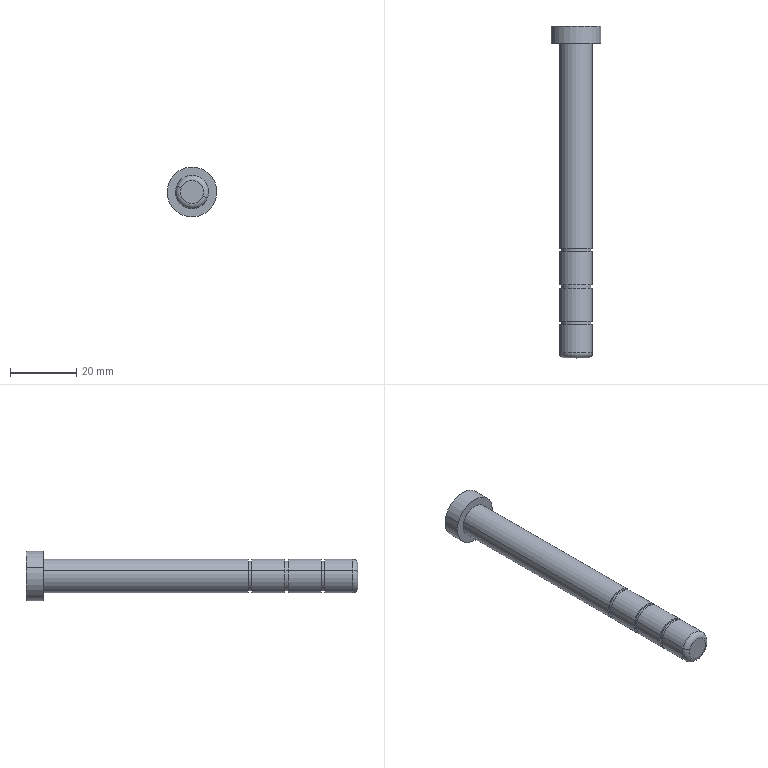Component | SolidWorks | GP-10-100-2GuidePin-2 | 1 solid | 27 faces | box 15 x 100 x 15 mm | volume 8306 mm3 | cylinder 16 | plane 9 | torus 2 | commonest cylinder face diameters 10 x8 9 x6 15 x2
build123d program:
from build123d import *

# Parameters (mm, degrees)
FILLET1_R = 1.5


with BuildPart() as part:
    # Sketch1 → Revolve1 (revolve)
    with BuildSketch(Plane.XY, mode=Mode.PRIVATE) as revolve1_sk:
        Polygon((0, 100), (5, 100), (5, 90), (4.5, 90), (4.5, 89), (5, 89), (5, 79), (4.5, 79), (4.5, 78), (5, 78), (5, 68), (4.5, 68), (4.5, 67), (5, 67), (5, 5.2), (7.5, 5.2), (7.5, 0), (0, 0), align=None)
    revolve(revolve1_sk.sketch.rotate(Axis((0, 100, 0), (0, -1, 0)), 180), axis=Axis((0, 100, 0), (0, -1, 0)))

    # Fillet1
    fillet1_edges = [part.edges().sort_by_distance(p)[0] for p in [
        (5, 100, 0),
    ]]
    fillet(fillet1_edges, radius=FILLET1_R)


solid = part.part

# Placed as in the assembly
solid = solid.moved(Location((139.884, -65.161, 270), (180, 0, 0)))
STEP:
#1=CARTESIAN_POINT('',(5.378,-6.502,10.677));
#2=VERTEX_POINT('',#1);
#3=CARTESIAN_POINT('',(5.637,-6.502,10.583));
#4=VERTEX_POINT('',#3);
#5=CARTESIAN_POINT('',(5.507,-6.502,10.63));
#6=DIRECTION('',(-0.,-1.,0.));
#7=DIRECTION('',(0.9396,0.,-0.3423));
#8=AXIS2_PLACEMENT_3D('',#5,#6,#7);
#9=CIRCLE('',#8,0.1378);
#10=EDGE_CURVE('',#2,#4,#9,.T.);
#11=ORIENTED_EDGE('',*,*,#10,.F.);
#12=CARTESIAN_POINT('',(5.322,-6.443,10.697));
#13=VERTEX_POINT('',#12);
#14=CARTESIAN_POINT('',(5.378,-6.443,10.677));
#15=DIRECTION('',(-0.3423,0.,-0.9396));
#16=DIRECTION('',(-0.9396,0.,0.3423));
#17=AXIS2_PLACEMENT_3D('',#14,#15,#16);
#18=CIRCLE('',#17,0.05906);
#19=EDGE_CURVE('',#2,#13,#18,.T.);
#20=ORIENTED_EDGE('',*,*,#19,.T.);
#21=CARTESIAN_POINT('',(5.692,-6.443,10.563));
#22=VERTEX_POINT('',#21);
#23=CARTESIAN_POINT('',(5.507,-6.443,10.63));
#24=DIRECTION('',(0.,1.,-0.));
#25=DIRECTION('',(0.9396,0.,-0.3423));
#26=AXIS2_PLACEMENT_3D('',#23,#24,#25);
#27=CIRCLE('',#26,0.1969);
#28=EDGE_CURVE('',#22,#13,#27,.T.);
#29=ORIENTED_EDGE('',*,*,#28,.F.);
#30=CARTESIAN_POINT('',(5.637,-6.443,10.583));
#31=DIRECTION('',(0.3423,-0.,0.9396));
#32=DIRECTION('',(0.9396,0.,-0.3423));
#33=AXIS2_PLACEMENT_3D('',#30,#31,#32);
#34=CIRCLE('',#33,0.05906);
#35=EDGE_CURVE('',#4,#22,#34,.T.);
#36=ORIENTED_EDGE('',*,*,#35,.F.);
#37=EDGE_LOOP('',(#11,#20,#29,#36));
#38=FACE_OUTER_BOUND('',#37,.T.);
#39=CARTESIAN_POINT('',(5.507,-6.443,10.63));
#40=DIRECTION('',(0.,1.,-0.));
#41=DIRECTION('',(0.9396,-0.,-0.3423));
#42=AXIS2_PLACEMENT_3D('',#39,#40,#41);
#43=TOROIDAL_SURFACE('',#42,0.1378,0.05906);
#44=ADVANCED_FACE('',(#38),#43,.T.);
#45=CARTESIAN_POINT('',(5.23,-2.565,10.731));
#46=VERTEX_POINT('',#45);
#47=CARTESIAN_POINT('',(5.785,-2.565,10.529));
#48=VERTEX_POINT('',#47);
#49=CARTESIAN_POINT('',(5.507,-2.565,10.63));
#50=DIRECTION('',(-0.,-1.,0.));
#51=DIRECTION('',(-0.9396,0.,0.3423));
#52=AXIS2_PLACEMENT_3D('',#49,#50,#51);
#53=CIRCLE('',#52,0.2953);
#54=EDGE_CURVE('',#46,#48,#53,.T.);
#55=ORIENTED_EDGE('',*,*,#54,.T.);
#56=CARTESIAN_POINT('',(5.785,-2.77,10.529));
#57=VERTEX_POINT('',#56);
#58=CARTESIAN_POINT('',(5.785,-6.502,10.529));
#59=DIRECTION('',(-0.,-1.,0.));
#60=VECTOR('',#59,39.37);
#61=LINE('',#58,#60);
#62=EDGE_CURVE('',#48,#57,#61,.T.);
#63=ORIENTED_EDGE('',*,*,#62,.T.);
#64=CARTESIAN_POINT('',(5.23,-2.77,10.731));
#65=VERTEX_POINT('',#64);
#66=CARTESIAN_POINT('',(5.507,-2.77,10.63));
#67=DIRECTION('',(-0.,-1.,0.));
#68=DIRECTION('',(-0.9396,0.,0.3423));
#69=AXIS2_PLACEMENT_3D('',#66,#67,#68);
#70=CIRCLE('',#69,0.2953);
#71=EDGE_CURVE('',#65,#57,#70,.T.);
#72=ORIENTED_EDGE('',*,*,#71,.F.);
#73=CARTESIAN_POINT('',(5.23,-6.502,10.731));
#74=DIRECTION('',(-0.,-1.,0.));
#75=VECTOR('',#74,39.37);
#76=LINE('',#73,#75);
#77=EDGE_CURVE('',#46,#65,#76,.T.);
#78=ORIENTED_EDGE('',*,*,#77,.F.);
#79=EDGE_LOOP('',(#55,#63,#72,#78));
#80=FACE_OUTER_BOUND('',#79,.T.);
#81=CARTESIAN_POINT('',(5.507,-6.502,10.63));
#82=DIRECTION('',(-0.,-1.,0.));
#83=DIRECTION('',(-0.9396,0.,0.3423));
#84=AXIS2_PLACEMENT_3D('',#81,#82,#83);
#85=CYLINDRICAL_SURFACE('',#84,0.2953);
#86=ADVANCED_FACE('',(#80),#85,.T.);
#87=CARTESIAN_POINT('',(5.322,-2.77,10.697));
#88=VERTEX_POINT('',#87);
#89=CARTESIAN_POINT('',(5.692,-2.77,10.563));
#90=VERTEX_POINT('',#89);
#91=CARTESIAN_POINT('',(5.507,-2.77,10.63));
#92=DIRECTION('',(-0.,-1.,0.));
#93=DIRECTION('',(-0.9396,0.,0.3423));
#94=AXIS2_PLACEMENT_3D('',#91,#92,#93);
#95=CIRCLE('',#94,0.1969);
#96=EDGE_CURVE('',#88,#90,#95,.T.);
#97=ORIENTED_EDGE('',*,*,#96,.T.);
#98=CARTESIAN_POINT('',(5.692,-5.203,10.563));
#99=VERTEX_POINT('',#98);
#100=CARTESIAN_POINT('',(5.692,-6.502,10.563));
#101=DIRECTION('',(-0.,-1.,0.));
#102=VECTOR('',#101,39.37);
#103=LINE('',#100,#102);
#104=EDGE_CURVE('',#90,#99,#103,.T.);
#105=ORIENTED_EDGE('',*,*,#104,.T.);
#106=CARTESIAN_POINT('',(5.322,-5.203,10.697));
#107=VERTEX_POINT('',#106);
#108=CARTESIAN_POINT('',(5.507,-5.203,10.63));
#109=DIRECTION('',(-0.,-1.,0.));
#110=DIRECTION('',(-0.9396,0.,0.3423));
#111=AXIS2_PLACEMENT_3D('',#108,#109,#110);
#112=CIRCLE('',#111,0.1969);
#113=EDGE_CURVE('',#107,#99,#112,.T.);
#114=ORIENTED_EDGE('',*,*,#113,.F.);
#115=CARTESIAN_POINT('',(5.322,-6.502,10.697));
#116=DIRECTION('',(-0.,-1.,0.));
#117=VECTOR('',#116,39.37);
#118=LINE('',#115,#117);
#119=EDGE_CURVE('',#88,#107,#118,.T.);
#120=ORIENTED_EDGE('',*,*,#119,.F.);
#121=EDGE_LOOP('',(#97,#105,#114,#120));
#122=FACE_OUTER_BOUND('',#121,.T.);
#123=CARTESIAN_POINT('',(5.507,-6.502,10.63));
#124=DIRECTION('',(-0.,-1.,0.));
#125=DIRECTION('',(-0.9396,0.,0.3423));
#126=AXIS2_PLACEMENT_3D('',#123,#124,#125);
#127=CYLINDRICAL_SURFACE('',#126,0.1969);
#128=ADVANCED_FACE('',(#122),#127,.T.);
#129=CARTESIAN_POINT('',(5.341,-5.203,10.691));
#130=VERTEX_POINT('',#129);
#131=CARTESIAN_POINT('',(5.674,-5.203,10.569));
#132=VERTEX_POINT('',#131);
#133=CARTESIAN_POINT('',(5.507,-5.203,10.63));
#134=DIRECTION('',(-0.,-1.,0.));
#135=DIRECTION('',(-0.9396,0.,0.3423));
#136=AXIS2_PLACEMENT_3D('',#133,#134,#135);
#137=CIRCLE('',#136,0.1772);
#138=EDGE_CURVE('',#130,#132,#137,.T.);
#139=ORIENTED_EDGE('',*,*,#138,.T.);
#140=CARTESIAN_POINT('',(5.674,-5.243,10.569));
#141=VERTEX_POINT('',#140);
#142=CARTESIAN_POINT('',(5.674,-6.502,10.569));
#143=DIRECTION('',(-0.,-1.,0.));
#144=VECTOR('',#143,39.37);
#145=LINE('',#142,#144);
#146=EDGE_CURVE('',#132,#141,#145,.T.);
#147=ORIENTED_EDGE('',*,*,#146,.T.);
#148=CARTESIAN_POINT('',(5.341,-5.243,10.691));
#149=VERTEX_POINT('',#148);
#150=CARTESIAN_POINT('',(5.507,-5.243,10.63));
#151=DIRECTION('',(-0.,-1.,0.));
#152=DIRECTION('',(-0.9396,0.,0.3423));
#153=AXIS2_PLACEMENT_3D('',#150,#151,#152);
#154=CIRCLE('',#153,0.1772);
#155=EDGE_CURVE('',#149,#141,#154,.T.);
#156=ORIENTED_EDGE('',*,*,#155,.F.);
#157=CARTESIAN_POINT('',(5.341,-6.502,10.691));
#158=DIRECTION('',(-0.,-1.,0.));
#159=VECTOR('',#158,39.37);
#160=LINE('',#157,#159);
#161=EDGE_CURVE('',#130,#149,#160,.T.);
#162=ORIENTED_EDGE('',*,*,#161,.F.);
#163=EDGE_LOOP('',(#139,#147,#156,#162));
#164=FACE_OUTER_BOUND('',#163,.T.);
#165=CARTESIAN_POINT('',(5.507,-6.502,10.63));
#166=DIRECTION('',(-0.,-1.,0.));
#167=DIRECTION('',(-0.9396,0.,0.3423));
#168=AXIS2_PLACEMENT_3D('',#165,#166,#167);
#169=CYLINDRICAL_SURFACE('',#168,0.1772);
#170=ADVANCED_FACE('',(#164),#169,.T.);
#171=CARTESIAN_POINT('',(5.322,-5.243,10.697));
#172=VERTEX_POINT('',#171);
#173=CARTESIAN_POINT('',(5.692,-5.243,10.563));
#174=VERTEX_POINT('',#173);
#175=CARTESIAN_POINT('',(5.507,-5.243,10.63));
#176=DIRECTION('',(-0.,-1.,0.));
#177=DIRECTION('',(-0.9396,0.,0.3423));
#178=AXIS2_PLACEMENT_3D('',#175,#176,#177);
#179=CIRCLE('',#178,0.1969);
#180=EDGE_CURVE('',#172,#174,#179,.T.);
#181=ORIENTED_EDGE('',*,*,#180,.T.);
#182=CARTESIAN_POINT('',(5.692,-5.636,10.563));
#183=VERTEX_POINT('',#182);
#184=CARTESIAN_POINT('',(5.692,-6.502,10.563));
#185=DIRECTION('',(-0.,-1.,0.));
#186=VECTOR('',#185,39.37);
#187=LINE('',#184,#186);
#188=EDGE_CURVE('',#174,#183,#187,.T.);
#189=ORIENTED_EDGE('',*,*,#188,.T.);
#190=CARTESIAN_POINT('',(5.322,-5.636,10.697));
#191=VERTEX_POINT('',#190);
#192=CARTESIAN_POINT('',(5.507,-5.636,10.63));
#193=DIRECTION('',(-0.,-1.,0.));
#194=DIRECTION('',(-0.9396,0.,0.3423));
#195=AXIS2_PLACEMENT_3D('',#192,#193,#194);
#196=CIRCLE('',#195,0.1969);
#197=EDGE_CURVE('',#191,#183,#196,.T.);
#198=ORIENTED_EDGE('',*,*,#197,.F.);
#199=CARTESIAN_POINT('',(5.322,-6.502,10.697));
#200=DIRECTION('',(-0.,-1.,0.));
#201=VECTOR('',#200,39.37);
#202=LINE('',#199,#201);
#203=EDGE_CURVE('',#172,#191,#202,.T.);
#204=ORIENTED_EDGE('',*,*,#203,.F.);
#205=EDGE_LOOP('',(#181,#189,#198,#204));
#206=FACE_OUTER_BOUND('',#205,.T.);
#207=CARTESIAN_POINT('',(5.507,-6.502,10.63));
#208=DIRECTION('',(-0.,-1.,0.));
#209=DIRECTION('',(-0.9396,0.,0.3423));
#210=AXIS2_PLACEMENT_3D('',#207,#208,#209);
#211=CYLINDRICAL_SURFACE('',#210,0.1969);
#212=ADVANCED_FACE('',(#206),#211,.T.);
#213=CARTESIAN_POINT('',(5.341,-5.636,10.691));
#214=VERTEX_POINT('',#213);
#215=CARTESIAN_POINT('',(5.674,-5.636,10.569));
#216=VERTEX_POINT('',#215);
#217=CARTESIAN_POINT('',(5.507,-5.636,10.63));
#218=DIRECTION('',(-0.,-1.,0.));
#219=DIRECTION('',(-0.9396,0.,0.3423));
#220=AXIS2_PLACEMENT_3D('',#217,#218,#219);
#221=CIRCLE('',#220,0.1772);
#222=EDGE_CURVE('',#214,#216,#221,.T.);
#223=ORIENTED_EDGE('',*,*,#222,.T.);
#224=CARTESIAN_POINT('',(5.674,-5.676,10.569));
#225=VERTEX_POINT('',#224);
#226=CARTESIAN_POINT('',(5.674,-6.502,10.569));
#227=DIRECTION('',(-0.,-1.,0.));
#228=VECTOR('',#227,39.37);
#229=LINE('',#226,#228);
#230=EDGE_CURVE('',#216,#225,#229,.T.);
#231=ORIENTED_EDGE('',*,*,#230,.T.);
#232=CARTESIAN_POINT('',(5.341,-5.676,10.691));
#233=VERTEX_POINT('',#232);
#234=CARTESIAN_POINT('',(5.507,-5.676,10.63));
#235=DIRECTION('',(-0.,-1.,0.));
#236=DIRECTION('',(-0.9396,0.,0.3423));
#237=AXIS2_PLACEMENT_3D('',#234,#235,#236);
#238=CIRCLE('',#237,0.1772);
#239=EDGE_CURVE('',#233,#225,#238,.T.);
#240=ORIENTED_EDGE('',*,*,#239,.F.);
#241=CARTESIAN_POINT('',(5.341,-6.502,10.691));
#242=DIRECTION('',(-0.,-1.,0.));
#243=VECTOR('',#242,39.37);
#244=LINE('',#241,#243);
#245=EDGE_CURVE('',#214,#233,#244,.T.);
#246=ORIENTED_EDGE('',*,*,#245,.F.);
#247=EDGE_LOOP('',(#223,#231,#240,#246));
#248=FACE_OUTER_BOUND('',#247,.T.);
#249=CARTESIAN_POINT('',(5.507,-6.502,10.63));
#250=DIRECTION('',(-0.,-1.,0.));
#251=DIRECTION('',(-0.9396,0.,0.3423));
#252=AXIS2_PLACEMENT_3D('',#249,#250,#251);
#253=CYLINDRICAL_SURFACE('',#252,0.1772);
#254=ADVANCED_FACE('',(#248),#253,.T.);
#255=CARTESIAN_POINT('',(5.322,-5.676,10.697));
#256=VERTEX_POINT('',#255);
#257=CARTESIAN_POINT('',(5.692,-5.676,10.563));
#258=VERTEX_POINT('',#257);
#259=CARTESIAN_POINT('',(5.507,-5.676,10.63));
#260=DIRECTION('',(-0.,-1.,0.));
#261=DIRECTION('',(-0.9396,0.,0.3423));
#262=AXIS2_PLACEMENT_3D('',#259,#260,#261);
#263=CIRCLE('',#262,0.1969);
#264=EDGE_CURVE('',#256,#258,#263,.T.);
#265=ORIENTED_EDGE('',*,*,#264,.T.);
#266=CARTESIAN_POINT('',(5.692,-6.069,10.563));
#267=VERTEX_POINT('',#266);
#268=CARTESIAN_POINT('',(5.692,-6.502,10.563));
#269=DIRECTION('',(-0.,-1.,0.));
#270=VECTOR('',#269,39.37);
#271=LINE('',#268,#270);
#272=EDGE_CURVE('',#258,#267,#271,.T.);
#273=ORIENTED_EDGE('',*,*,#272,.T.);
#274=CARTESIAN_POINT('',(5.322,-6.069,10.697));
#275=VERTEX_POINT('',#274);
#276=CARTESIAN_POINT('',(5.507,-6.069,10.63));
#277=DIRECTION('',(-0.,-1.,0.));
#278=DIRECTION('',(-0.9396,0.,0.3423));
#279=AXIS2_PLACEMENT_3D('',#276,#277,#278);
#280=CIRCLE('',#279,0.1969);
#281=EDGE_CURVE('',#275,#267,#280,.T.);
#282=ORIENTED_EDGE('',*,*,#281,.F.);
#283=CARTESIAN_POINT('',(5.322,-6.502,10.697));
#284=DIRECTION('',(-0.,-1.,0.));
#285=VECTOR('',#284,39.37);
#286=LINE('',#283,#285);
#287=EDGE_CURVE('',#256,#275,#286,.T.);
#288=ORIENTED_EDGE('',*,*,#287,.F.);
#289=EDGE_LOOP('',(#265,#273,#282,#288));
#290=FACE_OUTER_BOUND('',#289,.T.);
#291=CARTESIAN_POINT('',(5.507,-6.502,10.63));
#292=DIRECTION('',(-0.,-1.,0.));
#293=DIRECTION('',(-0.9396,0.,0.3423));
#294=AXIS2_PLACEMENT_3D('',#291,#292,#293);
#295=CYLINDRICAL_SURFACE('',#294,0.1969);
#296=ADVANCED_FACE('',(#290),#295,.T.);
#297=CARTESIAN_POINT('',(5.341,-6.069,10.691));
#298=VERTEX_POINT('',#297);
#299=CARTESIAN_POINT('',(5.674,-6.069,10.569));
#300=VERTEX_POINT('',#299);
#301=CARTESIAN_POINT('',(5.507,-6.069,10.63));
#302=DIRECTION('',(-0.,-1.,0.));
#303=DIRECTION('',(-0.9396,0.,0.3423));
#304=AXIS2_PLACEMENT_3D('',#301,#302,#303);
#305=CIRCLE('',#304,0.1772);
#306=EDGE_CURVE('',#298,#300,#305,.T.);
#307=ORIENTED_EDGE('',*,*,#306,.T.);
#308=CARTESIAN_POINT('',(5.674,-6.109,10.569));
#309=VERTEX_POINT('',#308);
#310=CARTESIAN_POINT('',(5.674,-6.502,10.569));
#311=DIRECTION('',(-0.,-1.,0.));
#312=VECTOR('',#311,39.37);
#313=LINE('',#310,#312);
#314=EDGE_CURVE('',#300,#309,#313,.T.);
#315=ORIENTED_EDGE('',*,*,#314,.T.);
#316=CARTESIAN_POINT('',(5.341,-6.109,10.691));
#317=VERTEX_POINT('',#316);
#318=CARTESIAN_POINT('',(5.507,-6.109,10.63));
#319=DIRECTION('',(-0.,-1.,0.));
#320=DIRECTION('',(-0.9396,0.,0.3423));
#321=AXIS2_PLACEMENT_3D('',#318,#319,#320);
#322=CIRCLE('',#321,0.1772);
#323=EDGE_CURVE('',#317,#309,#322,.T.);
#324=ORIENTED_EDGE('',*,*,#323,.F.);
#325=CARTESIAN_POINT('',(5.341,-6.502,10.691));
#326=DIRECTION('',(-0.,-1.,0.));
#327=VECTOR('',#326,39.37);
#328=LINE('',#325,#327);
#329=EDGE_CURVE('',#298,#317,#328,.T.);
#330=ORIENTED_EDGE('',*,*,#329,.F.);
#331=EDGE_LOOP('',(#307,#315,#324,#330));
#332=FACE_OUTER_BOUND('',#331,.T.);
#333=CARTESIAN_POINT('',(5.507,-6.502,10.63));
#334=DIRECTION('',(-0.,-1.,0.));
#335=DIRECTION('',(-0.9396,0.,0.3423));
#336=AXIS2_PLACEMENT_3D('',#333,#334,#335);
#337=CYLINDRICAL_SURFACE('',#336,0.1772);
#338=ADVANCED_FACE('',(#332),#337,.T.);
#339=CARTESIAN_POINT('',(5.322,-6.109,10.697));
#340=VERTEX_POINT('',#339);
#341=CARTESIAN_POINT('',(5.692,-6.109,10.563));
#342=VERTEX_POINT('',#341);
#343=CARTESIAN_POINT('',(5.507,-6.109,10.63));
#344=DIRECTION('',(-0.,-1.,0.));
#345=DIRECTION('',(-0.9396,0.,0.3423));
#346=AXIS2_PLACEMENT_3D('',#343,#344,#345);
#347=CIRCLE('',#346,0.1969);
#348=EDGE_CURVE('',#340,#342,#347,.T.);
#349=ORIENTED_EDGE('',*,*,#348,.T.);
#350=CARTESIAN_POINT('',(5.692,-6.502,10.563));
#351=DIRECTION('',(-0.,-1.,0.));
#352=VECTOR('',#351,39.37);
#353=LINE('',#350,#352);
#354=EDGE_CURVE('',#342,#22,#353,.T.);
#355=ORIENTED_EDGE('',*,*,#354,.T.);
#356=ORIENTED_EDGE('',*,*,#28,.T.);
#357=CARTESIAN_POINT('',(5.322,-6.502,10.697));
#358=DIRECTION('',(-0.,-1.,0.));
#359=VECTOR('',#358,39.37);
#360=LINE('',#357,#359);
#361=EDGE_CURVE('',#340,#13,#360,.T.);
#362=ORIENTED_EDGE('',*,*,#361,.F.);
#363=EDGE_LOOP('',(#349,#355,#356,#362));
#364=FACE_OUTER_BOUND('',#363,.T.);
#365=CARTESIAN_POINT('',(5.507,-6.502,10.63));
#366=DIRECTION('',(-0.,-1.,0.));
#367=DIRECTION('',(-0.9396,0.,0.3423));
#368=AXIS2_PLACEMENT_3D('',#365,#366,#367);
#369=CYLINDRICAL_SURFACE('',#368,0.1969);
#370=ADVANCED_FACE('',(#364),#369,.T.);
#371=CARTESIAN_POINT('',(5.507,-6.502,10.63));
#372=DIRECTION('',(-0.,-1.,0.));
#373=DIRECTION('',(0.9396,0.,-0.3423));
#374=AXIS2_PLACEMENT_3D('',#371,#372,#373);
#375=CIRCLE('',#374,0.1378);
#376=EDGE_CURVE('',#4,#2,#375,.T.);
#377=ORIENTED_EDGE('',*,*,#376,.T.);
#378=ORIENTED_EDGE('',*,*,#10,.T.);
#379=EDGE_LOOP('',(#377,#378));
#380=FACE_OUTER_BOUND('',#379,.T.);
#381=CARTESIAN_POINT('',(5.507,-6.502,10.63));
#382=DIRECTION('',(0.,1.,-0.));
#383=DIRECTION('',(0.9396,-0.,-0.3423));
#384=AXIS2_PLACEMENT_3D('',#381,#382,#383);
#385=PLANE('',#384);
#386=ADVANCED_FACE('',(#380),#385,.F.);
#387=ORIENTED_EDGE('',*,*,#354,.F.);
#388=CARTESIAN_POINT('',(5.507,-6.109,10.63));
#389=DIRECTION('',(-0.,-1.,0.));
#390=DIRECTION('',(-0.9396,0.,0.3423));
#391=AXIS2_PLACEMENT_3D('',#388,#389,#390);
#392=CIRCLE('',#391,0.1969);
#393=EDGE_CURVE('',#342,#340,#392,.T.);
#394=ORIENTED_EDGE('',*,*,#393,.T.);
#395=ORIENTED_EDGE('',*,*,#361,.T.);
#396=CARTESIAN_POINT('',(5.507,-6.443,10.63));
#397=DIRECTION('',(0.,1.,-0.));
#398=DIRECTION('',(0.9396,0.,-0.3423));
#399=AXIS2_PLACEMENT_3D('',#396,#397,#398);
#400=CIRCLE('',#399,0.1969);
#401=EDGE_CURVE('',#13,#22,#400,.T.);
#402=ORIENTED_EDGE('',*,*,#401,.T.);
#403=EDGE_LOOP('',(#387,#394,#395,#402));
#404=FACE_OUTER_BOUND('',#403,.T.);
#405=CARTESIAN_POINT('',(5.507,-6.502,10.63));
#406=DIRECTION('',(-0.,-1.,0.));
#407=DIRECTION('',(-0.9396,0.,0.3423));
#408=AXIS2_PLACEMENT_3D('',#405,#406,#407);
#409=CYLINDRICAL_SURFACE('',#408,0.1969);
#410=ADVANCED_FACE('',(#404),#409,.T.);
#411=ORIENTED_EDGE('',*,*,#348,.F.);
#412=ORIENTED_EDGE('',*,*,#393,.F.);
#413=EDGE_LOOP('',(#411,#412));
#414=FACE_OUTER_BOUND('',#413,.T.);
#415=ORIENTED_EDGE('',*,*,#323,.T.);
#416=CARTESIAN_POINT('',(5.507,-6.109,10.63));
#417=DIRECTION('',(-0.,-1.,0.));
#418=DIRECTION('',(-0.9396,0.,0.3423));
#419=AXIS2_PLACEMENT_3D('',#416,#417,#418);
#420=CIRCLE('',#419,0.1772);
#421=EDGE_CURVE('',#309,#317,#420,.T.);
#422=ORIENTED_EDGE('',*,*,#421,.T.);
#423=EDGE_LOOP('',(#415,#422));
#424=FACE_BOUND('',#423,.T.);
#425=CARTESIAN_POINT('',(5.692,-6.109,10.563));
#426=DIRECTION('',(-0.,-1.,0.));
#427=DIRECTION('',(-0.9396,0.,0.3423));
#428=AXIS2_PLACEMENT_3D('',#425,#426,#427);
#429=PLANE('',#428);
#430=ADVANCED_FACE('',(#414,#424),#429,.F.);
#431=ORIENTED_EDGE('',*,*,#314,.F.);
#432=CARTESIAN_POINT('',(5.507,-6.069,10.63));
#433=DIRECTION('',(-0.,-1.,0.));
#434=DIRECTION('',(-0.9396,0.,0.3423));
#435=AXIS2_PLACEMENT_3D('',#432,#433,#434);
#436=CIRCLE('',#435,0.1772);
#437=EDGE_CURVE('',#300,#298,#436,.T.);
#438=ORIENTED_EDGE('',*,*,#437,.T.);
#439=ORIENTED_EDGE('',*,*,#329,.T.);
#440=ORIENTED_EDGE('',*,*,#421,.F.);
#441=EDGE_LOOP('',(#431,#438,#439,#440));
#442=FACE_OUTER_BOUND('',#441,.T.);
#443=CARTESIAN_POINT('',(5.507,-6.502,10.63));
#444=DIRECTION('',(-0.,-1.,0.));
#445=DIRECTION('',(-0.9396,0.,0.3423));
#446=AXIS2_PLACEMENT_3D('',#443,#444,#445);
#447=CYLINDRICAL_SURFACE('',#446,0.1772);
#448=ADVANCED_FACE('',(#442),#447,.T.);
#449=ORIENTED_EDGE('',*,*,#306,.F.);
#450=ORIENTED_EDGE('',*,*,#437,.F.);
#451=EDGE_LOOP('',(#449,#450));
#452=FACE_BOUND('',#451,.T.);
#453=ORIENTED_EDGE('',*,*,#281,.T.);
#454=CARTESIAN_POINT('',(5.507,-6.069,10.63));
#455=DIRECTION('',(-0.,-1.,0.));
#456=DIRECTION('',(-0.9396,0.,0.3423));
#457=AXIS2_PLACEMENT_3D('',#454,#455,#456);
#458=CIRCLE('',#457,0.1969);
#459=EDGE_CURVE('',#267,#275,#458,.T.);
#460=ORIENTED_EDGE('',*,*,#459,.T.);
#461=EDGE_LOOP('',(#453,#460));
#462=FACE_OUTER_BOUND('',#461,.T.);
#463=CARTESIAN_POINT('',(5.674,-6.069,10.569));
#464=DIRECTION('',(0.,1.,-0.));
#465=DIRECTION('',(0.9396,-0.,-0.3423));
#466=AXIS2_PLACEMENT_3D('',#463,#464,#465);
#467=PLANE('',#466);
#468=ADVANCED_FACE('',(#452,#462),#467,.F.);
#469=ORIENTED_EDGE('',*,*,#272,.F.);
#470=CARTESIAN_POINT('',(5.507,-5.676,10.63));
#471=DIRECTION('',(-0.,-1.,0.));
#472=DIRECTION('',(-0.9396,0.,0.3423));
#473=AXIS2_PLACEMENT_3D('',#470,#471,#472);
#474=CIRCLE('',#473,0.1969);
#475=EDGE_CURVE('',#258,#256,#474,.T.);
#476=ORIENTED_EDGE('',*,*,#475,.T.);
#477=ORIENTED_EDGE('',*,*,#287,.T.);
#478=ORIENTED_EDGE('',*,*,#459,.F.);
#479=EDGE_LOOP('',(#469,#476,#477,#478));
#480=FACE_OUTER_BOUND('',#479,.T.);
#481=CARTESIAN_POINT('',(5.507,-6.502,10.63));
#482=DIRECTION('',(-0.,-1.,0.));
#483=DIRECTION('',(-0.9396,0.,0.3423));
#484=AXIS2_PLACEMENT_3D('',#481,#482,#483);
#485=CYLINDRICAL_SURFACE('',#484,0.1969);
#486=ADVANCED_FACE('',(#480),#485,.T.);
#487=ORIENTED_EDGE('',*,*,#264,.F.);
#488=ORIENTED_EDGE('',*,*,#475,.F.);
#489=EDGE_LOOP('',(#487,#488));
#490=FACE_OUTER_BOUND('',#489,.T.);
#491=ORIENTED_EDGE('',*,*,#239,.T.);
#492=CARTESIAN_POINT('',(5.507,-5.676,10.63));
#493=DIRECTION('',(-0.,-1.,0.));
#494=DIRECTION('',(-0.9396,0.,0.3423));
#495=AXIS2_PLACEMENT_3D('',#492,#493,#494);
#496=CIRCLE('',#495,0.1772);
#497=EDGE_CURVE('',#225,#233,#496,.T.);
#498=ORIENTED_EDGE('',*,*,#497,.T.);
#499=EDGE_LOOP('',(#491,#498));
#500=FACE_BOUND('',#499,.T.);
#501=CARTESIAN_POINT('',(5.692,-5.676,10.563));
#502=DIRECTION('',(-0.,-1.,0.));
#503=DIRECTION('',(-0.9396,0.,0.3423));
#504=AXIS2_PLACEMENT_3D('',#501,#502,#503);
#505=PLANE('',#504);
#506=ADVANCED_FACE('',(#490,#500),#505,.F.);
#507=ORIENTED_EDGE('',*,*,#230,.F.);
#508=CARTESIAN_POINT('',(5.507,-5.636,10.63));
#509=DIRECTION('',(-0.,-1.,0.));
#510=DIRECTION('',(-0.9396,0.,0.3423));
#511=AXIS2_PLACEMENT_3D('',#508,#509,#510);
#512=CIRCLE('',#511,0.1772);
#513=EDGE_CURVE('',#216,#214,#512,.T.);
#514=ORIENTED_EDGE('',*,*,#513,.T.);
#515=ORIENTED_EDGE('',*,*,#245,.T.);
#516=ORIENTED_EDGE('',*,*,#497,.F.);
#517=EDGE_LOOP('',(#507,#514,#515,#516));
#518=FACE_OUTER_BOUND('',#517,.T.);
#519=CARTESIAN_POINT('',(5.507,-6.502,10.63));
#520=DIRECTION('',(-0.,-1.,0.));
#521=DIRECTION('',(-0.9396,0.,0.3423));
#522=AXIS2_PLACEMENT_3D('',#519,#520,#521);
#523=CYLINDRICAL_SURFACE('',#522,0.1772);
#524=ADVANCED_FACE('',(#518),#523,.T.);
#525=ORIENTED_EDGE('',*,*,#222,.F.);
#526=ORIENTED_EDGE('',*,*,#513,.F.);
#527=EDGE_LOOP('',(#525,#526));
#528=FACE_BOUND('',#527,.T.);
#529=ORIENTED_EDGE('',*,*,#197,.T.);
#530=CARTESIAN_POINT('',(5.507,-5.636,10.63));
#531=DIRECTION('',(-0.,-1.,0.));
#532=DIRECTION('',(-0.9396,0.,0.3423));
#533=AXIS2_PLACEMENT_3D('',#530,#531,#532);
#534=CIRCLE('',#533,0.1969);
#535=EDGE_CURVE('',#183,#191,#534,.T.);
#536=ORIENTED_EDGE('',*,*,#535,.T.);
#537=EDGE_LOOP('',(#529,#536));
#538=FACE_OUTER_BOUND('',#537,.T.);
#539=CARTESIAN_POINT('',(5.674,-5.636,10.569));
#540=DIRECTION('',(0.,1.,-0.));
#541=DIRECTION('',(0.9396,-0.,-0.3423));
#542=AXIS2_PLACEMENT_3D('',#539,#540,#541);
#543=PLANE('',#542);
#544=ADVANCED_FACE('',(#528,#538),#543,.F.);
#545=ORIENTED_EDGE('',*,*,#188,.F.);
#546=CARTESIAN_POINT('',(5.507,-5.243,10.63));
#547=DIRECTION('',(-0.,-1.,0.));
#548=DIRECTION('',(-0.9396,0.,0.3423));
#549=AXIS2_PLACEMENT_3D('',#546,#547,#548);
#550=CIRCLE('',#549,0.1969);
#551=EDGE_CURVE('',#174,#172,#550,.T.);
#552=ORIENTED_EDGE('',*,*,#551,.T.);
#553=ORIENTED_EDGE('',*,*,#203,.T.);
#554=ORIENTED_EDGE('',*,*,#535,.F.);
#555=EDGE_LOOP('',(#545,#552,#553,#554));
#556=FACE_OUTER_BOUND('',#555,.T.);
#557=CARTESIAN_POINT('',(5.507,-6.502,10.63));
#558=DIRECTION('',(-0.,-1.,0.));
#559=DIRECTION('',(-0.9396,0.,0.3423));
#560=AXIS2_PLACEMENT_3D('',#557,#558,#559);
#561=CYLINDRICAL_SURFACE('',#560,0.1969);
#562=ADVANCED_FACE('',(#556),#561,.T.);
#563=ORIENTED_EDGE('',*,*,#180,.F.);
#564=ORIENTED_EDGE('',*,*,#551,.F.);
#565=EDGE_LOOP('',(#563,#564));
#566=FACE_OUTER_BOUND('',#565,.T.);
#567=ORIENTED_EDGE('',*,*,#155,.T.);
#568=CARTESIAN_POINT('',(5.507,-5.243,10.63));
#569=DIRECTION('',(-0.,-1.,0.));
#570=DIRECTION('',(-0.9396,0.,0.3423));
#571=AXIS2_PLACEMENT_3D('',#568,#569,#570);
#572=CIRCLE('',#571,0.1772);
#573=EDGE_CURVE('',#141,#149,#572,.T.);
#574=ORIENTED_EDGE('',*,*,#573,.T.);
#575=EDGE_LOOP('',(#567,#574));
#576=FACE_BOUND('',#575,.T.);
#577=CARTESIAN_POINT('',(5.692,-5.243,10.563));
#578=DIRECTION('',(-0.,-1.,0.));
#579=DIRECTION('',(-0.9396,0.,0.3423));
#580=AXIS2_PLACEMENT_3D('',#577,#578,#579);
#581=PLANE('',#580);
#582=ADVANCED_FACE('',(#566,#576),#581,.F.);
#583=ORIENTED_EDGE('',*,*,#146,.F.);
#584=CARTESIAN_POINT('',(5.507,-5.203,10.63));
#585=DIRECTION('',(-0.,-1.,0.));
#586=DIRECTION('',(-0.9396,0.,0.3423));
#587=AXIS2_PLACEMENT_3D('',#584,#585,#586);
#588=CIRCLE('',#587,0.1772);
#589=EDGE_CURVE('',#132,#130,#588,.T.);
#590=ORIENTED_EDGE('',*,*,#589,.T.);
#591=ORIENTED_EDGE('',*,*,#161,.T.);
#592=ORIENTED_EDGE('',*,*,#573,.F.);
#593=EDGE_LOOP('',(#583,#590,#591,#592));
#594=FACE_OUTER_BOUND('',#593,.T.);
#595=CARTESIAN_POINT('',(5.507,-6.502,10.63));
#596=DIRECTION('',(-0.,-1.,0.));
#597=DIRECTION('',(-0.9396,0.,0.3423));
#598=AXIS2_PLACEMENT_3D('',#595,#596,#597);
#599=CYLINDRICAL_SURFACE('',#598,0.1772);
#600=ADVANCED_FACE('',(#594),#599,.T.);
#601=ORIENTED_EDGE('',*,*,#138,.F.);
#602=ORIENTED_EDGE('',*,*,#589,.F.);
#603=EDGE_LOOP('',(#601,#602));
#604=FACE_BOUND('',#603,.T.);
#605=ORIENTED_EDGE('',*,*,#113,.T.);
#606=CARTESIAN_POINT('',(5.507,-5.203,10.63));
#607=DIRECTION('',(-0.,-1.,0.));
#608=DIRECTION('',(-0.9396,0.,0.3423));
#609=AXIS2_PLACEMENT_3D('',#606,#607,#608);
#610=CIRCLE('',#609,0.1969);
#611=EDGE_CURVE('',#99,#107,#610,.T.);
#612=ORIENTED_EDGE('',*,*,#611,.T.);
#613=EDGE_LOOP('',(#605,#612));
#614=FACE_OUTER_BOUND('',#613,.T.);
#615=CARTESIAN_POINT('',(5.674,-5.203,10.569));
#616=DIRECTION('',(0.,1.,-0.));
#617=DIRECTION('',(0.9396,-0.,-0.3423));
#618=AXIS2_PLACEMENT_3D('',#615,#616,#617);
#619=PLANE('',#618);
#620=ADVANCED_FACE('',(#604,#614),#619,.F.);
#621=ORIENTED_EDGE('',*,*,#104,.F.);
#622=CARTESIAN_POINT('',(5.507,-2.77,10.63));
#623=DIRECTION('',(-0.,-1.,0.));
#624=DIRECTION('',(-0.9396,0.,0.3423));
#625=AXIS2_PLACEMENT_3D('',#622,#623,#624);
#626=CIRCLE('',#625,0.1969);
#627=EDGE_CURVE('',#90,#88,#626,.T.);
#628=ORIENTED_EDGE('',*,*,#627,.T.);
#629=ORIENTED_EDGE('',*,*,#119,.T.);
#630=ORIENTED_EDGE('',*,*,#611,.F.);
#631=EDGE_LOOP('',(#621,#628,#629,#630));
#632=FACE_OUTER_BOUND('',#631,.T.);
#633=CARTESIAN_POINT('',(5.507,-6.502,10.63));
#634=DIRECTION('',(-0.,-1.,0.));
#635=DIRECTION('',(-0.9396,0.,0.3423));
#636=AXIS2_PLACEMENT_3D('',#633,#634,#635);
#637=CYLINDRICAL_SURFACE('',#636,0.1969);
#638=ADVANCED_FACE('',(#632),#637,.T.);
#639=ORIENTED_EDGE('',*,*,#96,.F.);
#640=ORIENTED_EDGE('',*,*,#627,.F.);
#641=EDGE_LOOP('',(#639,#640));
#642=FACE_BOUND('',#641,.T.);
#643=ORIENTED_EDGE('',*,*,#71,.T.);
#644=CARTESIAN_POINT('',(5.507,-2.77,10.63));
#645=DIRECTION('',(-0.,-1.,0.));
#646=DIRECTION('',(-0.9396,0.,0.3423));
#647=AXIS2_PLACEMENT_3D('',#644,#645,#646);
#648=CIRCLE('',#647,0.2953);
#649=EDGE_CURVE('',#57,#65,#648,.T.);
#650=ORIENTED_EDGE('',*,*,#649,.T.);
#651=EDGE_LOOP('',(#643,#650));
#652=FACE_OUTER_BOUND('',#651,.T.);
#653=CARTESIAN_POINT('',(5.692,-2.77,10.563));
#654=DIRECTION('',(0.,1.,-0.));
#655=DIRECTION('',(0.9396,-0.,-0.3423));
#656=AXIS2_PLACEMENT_3D('',#653,#654,#655);
#657=PLANE('',#656);
#658=ADVANCED_FACE('',(#642,#652),#657,.F.);
#659=ORIENTED_EDGE('',*,*,#62,.F.);
#660=CARTESIAN_POINT('',(5.507,-2.565,10.63));
#661=DIRECTION('',(-0.,-1.,0.));
#662=DIRECTION('',(-0.9396,0.,0.3423));
#663=AXIS2_PLACEMENT_3D('',#660,#661,#662);
#664=CIRCLE('',#663,0.2953);
#665=EDGE_CURVE('',#48,#46,#664,.T.);
#666=ORIENTED_EDGE('',*,*,#665,.T.);
#667=ORIENTED_EDGE('',*,*,#77,.T.);
#668=ORIENTED_EDGE('',*,*,#649,.F.);
#669=EDGE_LOOP('',(#659,#666,#667,#668));
#670=FACE_OUTER_BOUND('',#669,.T.);
#671=CARTESIAN_POINT('',(5.507,-6.502,10.63));
#672=DIRECTION('',(-0.,-1.,0.));
#673=DIRECTION('',(-0.9396,0.,0.3423));
#674=AXIS2_PLACEMENT_3D('',#671,#672,#673);
#675=CYLINDRICAL_SURFACE('',#674,0.2953);
#676=ADVANCED_FACE('',(#670),#675,.T.);
#677=ORIENTED_EDGE('',*,*,#54,.F.);
#678=ORIENTED_EDGE('',*,*,#665,.F.);
#679=EDGE_LOOP('',(#677,#678));
#680=FACE_OUTER_BOUND('',#679,.T.);
#681=CARTESIAN_POINT('',(5.785,-2.565,10.529));
#682=DIRECTION('',(-0.,-1.,0.));
#683=DIRECTION('',(-0.9396,0.,0.3423));
#684=AXIS2_PLACEMENT_3D('',#681,#682,#683);
#685=PLANE('',#684);
#686=ADVANCED_FACE('',(#680),#685,.F.);
#687=ORIENTED_EDGE('',*,*,#19,.F.);
#688=ORIENTED_EDGE('',*,*,#376,.F.);
#689=ORIENTED_EDGE('',*,*,#35,.T.);
#690=ORIENTED_EDGE('',*,*,#401,.F.);
#691=EDGE_LOOP('',(#687,#688,#689,#690));
#692=FACE_OUTER_BOUND('',#691,.T.);
#693=CARTESIAN_POINT('',(5.507,-6.443,10.63));
#694=DIRECTION('',(0.,1.,-0.));
#695=DIRECTION('',(0.9396,-0.,-0.3423));
#696=AXIS2_PLACEMENT_3D('',#693,#694,#695);
#697=TOROIDAL_SURFACE('',#696,0.1378,0.05906);
#698=ADVANCED_FACE('',(#692),#697,.T.);
#699=CLOSED_SHELL('',(#44,#86,#128,#170,#212,#254,#296,#338,#370,#386,#410,#430,#448,#468,#486,#506,#524,#544,#562,#582,#600,#620,#638,#658,#676,#686,#698));
#700=MANIFOLD_SOLID_BREP('',#699);
#701=CARTESIAN_POINT('',(0.,0.,0.));
#702=DIRECTION('',(0.,0.,1.));
#703=DIRECTION('',(1.,0.,0.));
#704=AXIS2_PLACEMENT_3D('',#701,#702,#703);
#705=(LENGTH_UNIT()NAMED_UNIT(*)SI_UNIT($,.METRE.));
#706=LENGTH_MEASURE_WITH_UNIT(LENGTH_MEASURE(0.0254),#705);
#707=DIMENSIONAL_EXPONENTS(1.,0.,0.,0.,0.,0.,0.);
#708=(CONVERSION_BASED_UNIT('',#706)LENGTH_UNIT()NAMED_UNIT(#707));
#709=UNCERTAINTY_MEASURE_WITH_UNIT(LENGTH_MEASURE(0.00001),#708,'','');
#710=(NAMED_UNIT(*)PLANE_ANGLE_UNIT()SI_UNIT($,.RADIAN.));
#711=(NAMED_UNIT(*)SI_UNIT($,.STERADIAN.)SOLID_ANGLE_UNIT());
#712=(GEOMETRIC_REPRESENTATION_CONTEXT(3)GLOBAL_UNCERTAINTY_ASSIGNED_CONTEXT((#709))GLOBAL_UNIT_ASSIGNED_CONTEXT((#708,#710,#711))REPRESENTATION_CONTEXT('',''));
#713=ADVANCED_BREP_SHAPE_REPRESENTATION('',(#700,#704),#712);
#714=COLOUR_RGB('',0.7922,0.8196,0.9333);
#715=FILL_AREA_STYLE_COLOUR('',#714);
#716=FILL_AREA_STYLE('',(#715));
#717=SURFACE_STYLE_FILL_AREA(#716);
#718=SURFACE_SIDE_STYLE('',(#717));
#719=SURFACE_STYLE_USAGE(.BOTH.,#718);
#720=PRESENTATION_STYLE_ASSIGNMENT((#719));
#721=STYLED_ITEM('',(#720),#700);
#722=(LENGTH_UNIT()NAMED_UNIT(*)SI_UNIT($,.METRE.));
#723=LENGTH_MEASURE_WITH_UNIT(LENGTH_MEASURE(0.0254),#722);
#724=DIMENSIONAL_EXPONENTS(1.,0.,0.,0.,0.,0.,0.);
#725=(CONVERSION_BASED_UNIT('',#723)LENGTH_UNIT()NAMED_UNIT(#724));
#726=UNCERTAINTY_MEASURE_WITH_UNIT(LENGTH_MEASURE(0.00001),#725,'','');
#727=(NAMED_UNIT(*)PLANE_ANGLE_UNIT()SI_UNIT($,.RADIAN.));
#728=(NAMED_UNIT(*)SI_UNIT($,.STERADIAN.)SOLID_ANGLE_UNIT());
#729=(GEOMETRIC_REPRESENTATION_CONTEXT(3)GLOBAL_UNCERTAINTY_ASSIGNED_CONTEXT((#726))GLOBAL_UNIT_ASSIGNED_CONTEXT((#725,#727,#728))REPRESENTATION_CONTEXT('',''));
#730=MECHANICAL_DESIGN_GEOMETRIC_PRESENTATION_REPRESENTATION('',(#721),#729);
#731=PRESENTATION_LAYER_ASSIGNMENT('','',(#721));